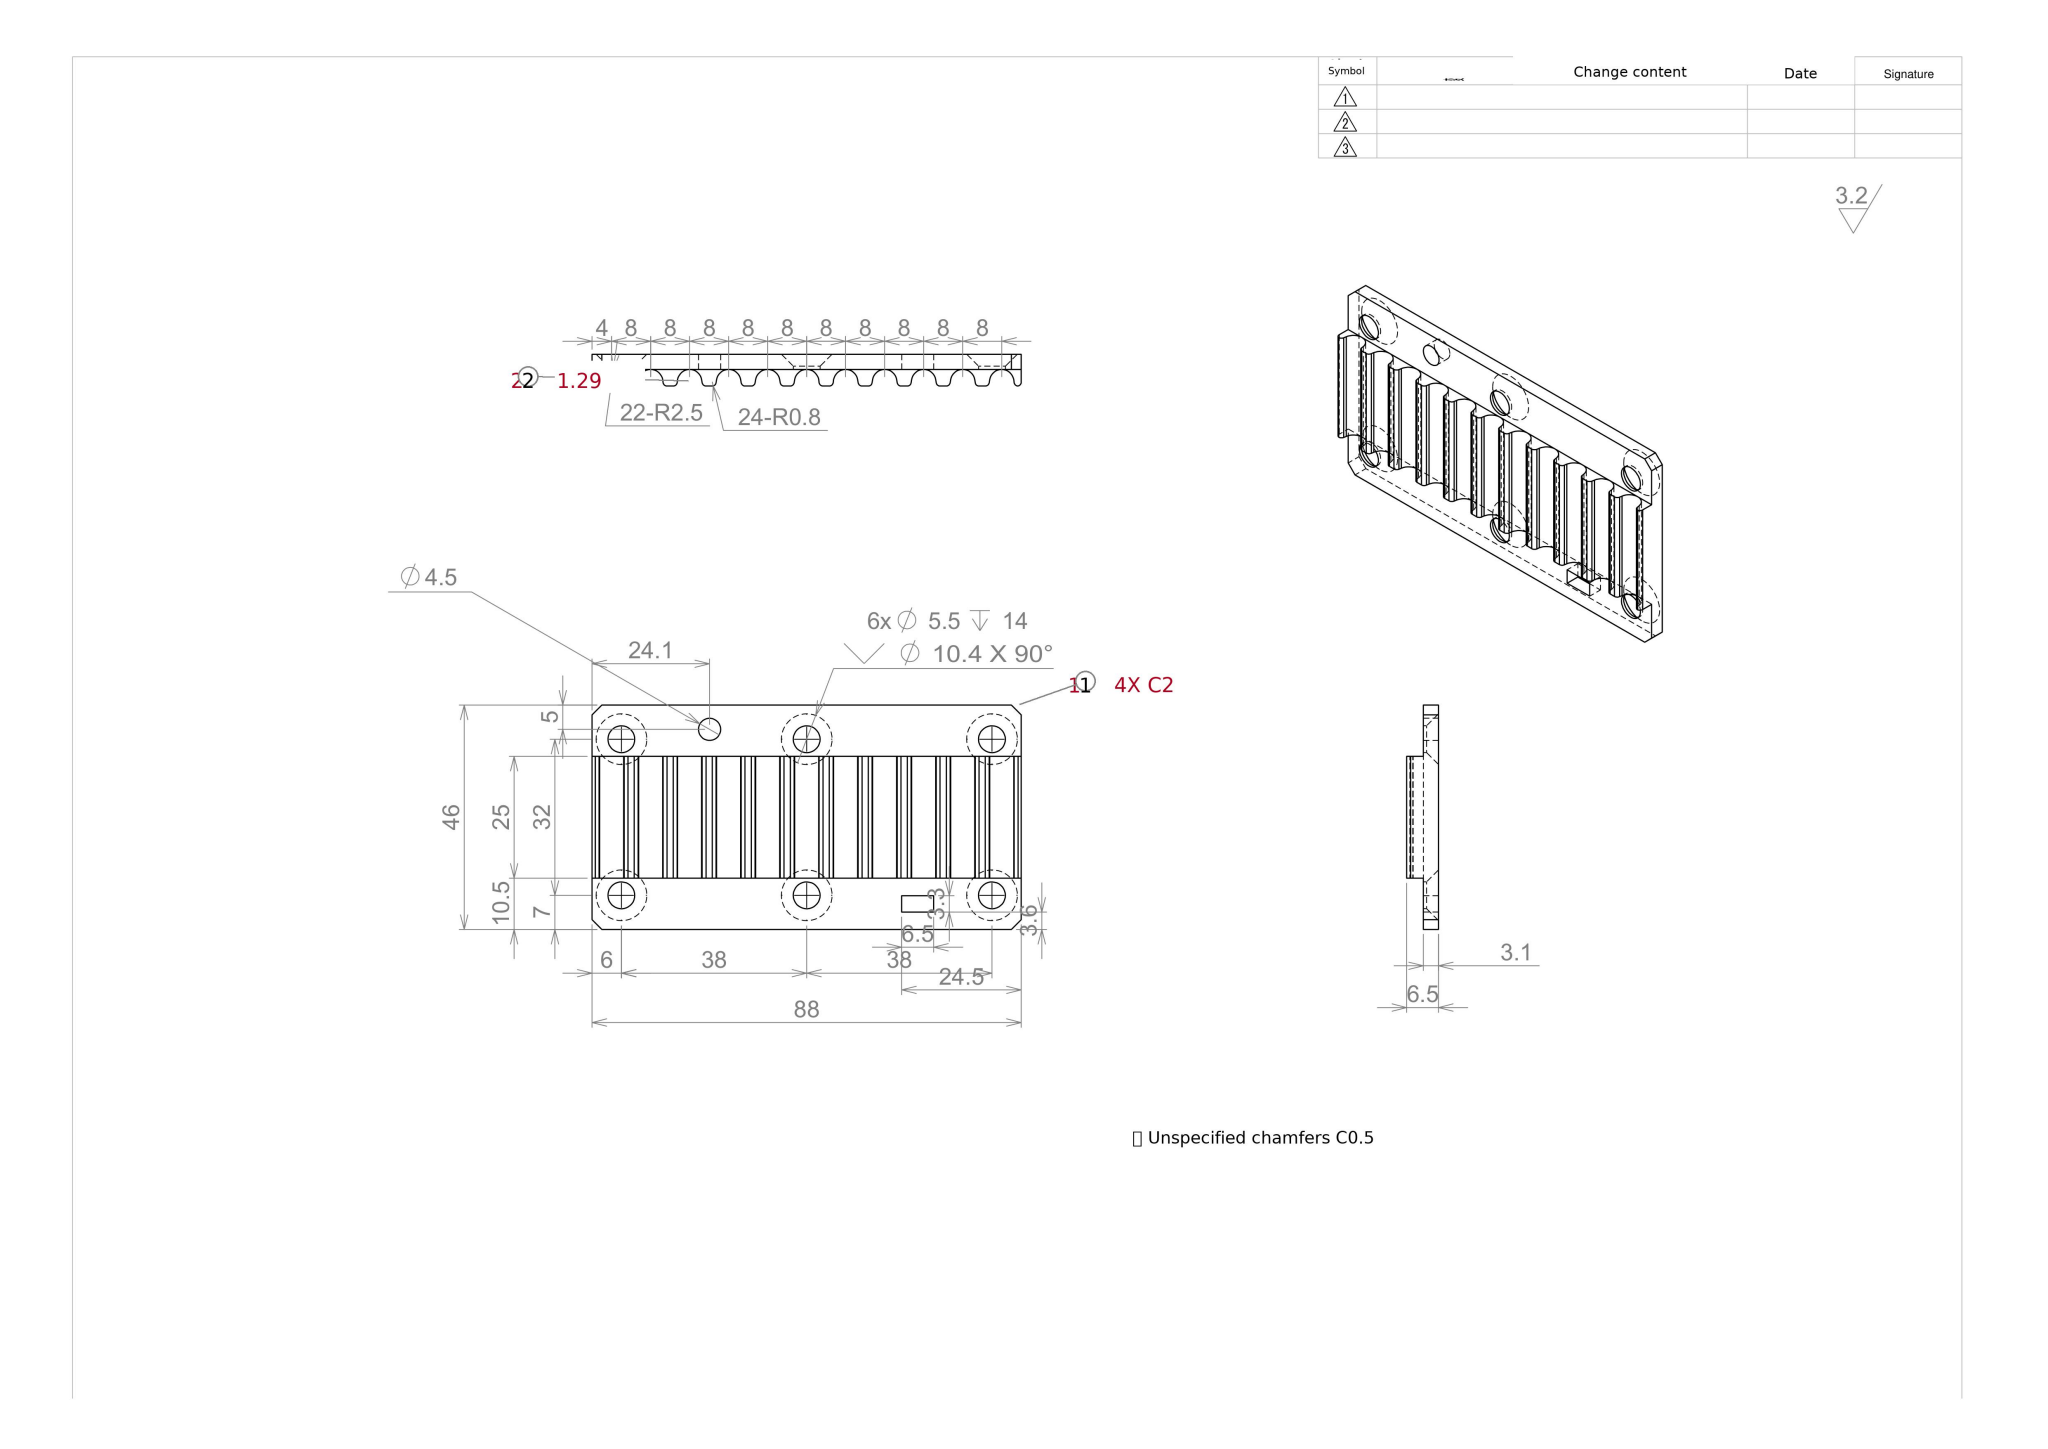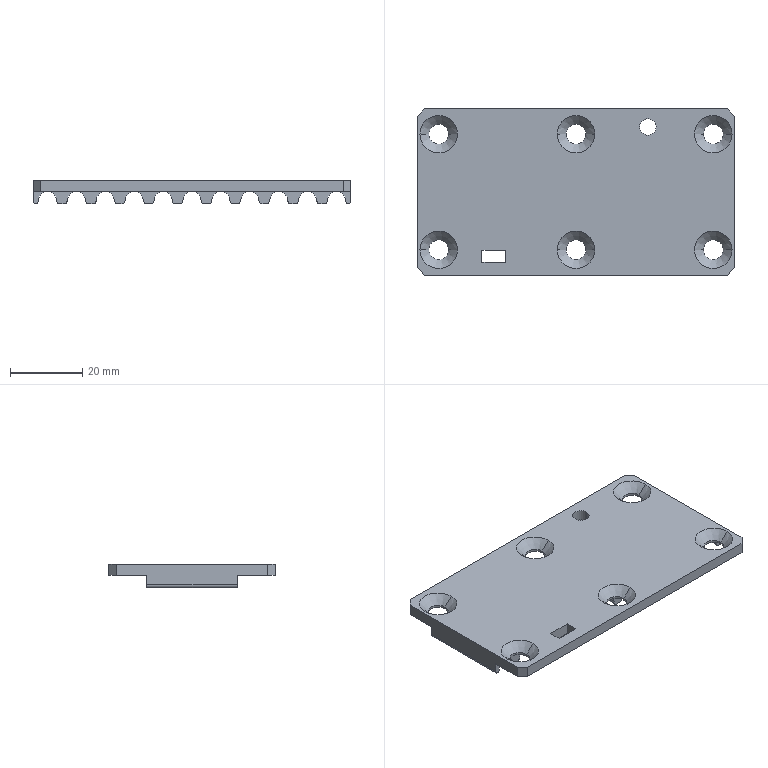Part | SolidWorks | mm | 1 solid | 132 faces | box 88 x 46 x 6.5 mm | volume 14992 mm3 | plane 71 | cylinder 49 | cone 12 | commonest cylinder face diameters 1.6 x24 5.5 x12 5 x11 4.547 x2